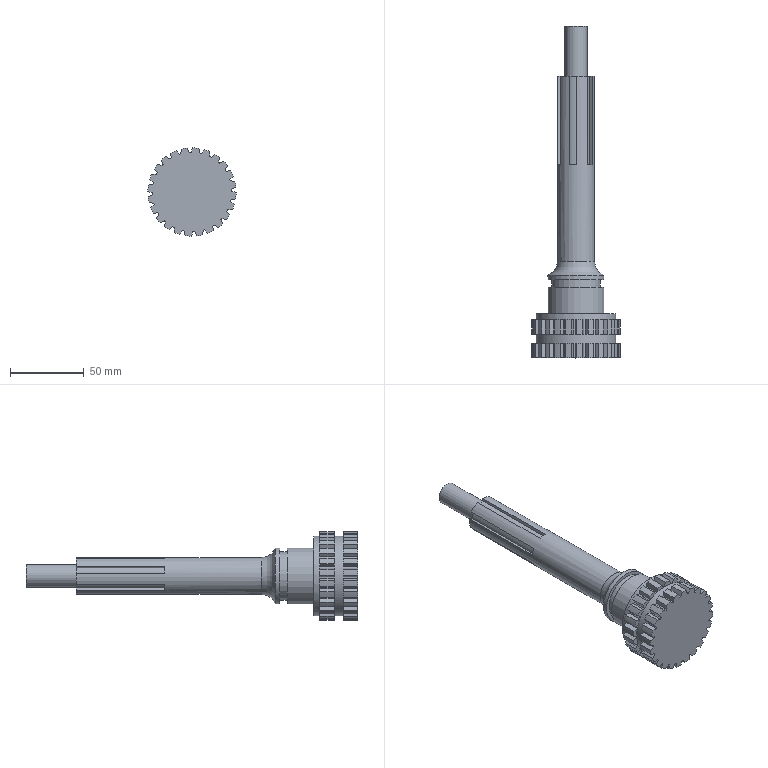Component | NX | DRIVE_SHAFT | 1 solid | 253 faces | volume 173232 mm3 | plane 192 | cylinder 60 | torus 1 | commonest cylinder face diameters 60 x48 20 x6 38 x2 25 x1 54 x1 33 x1 15 x1